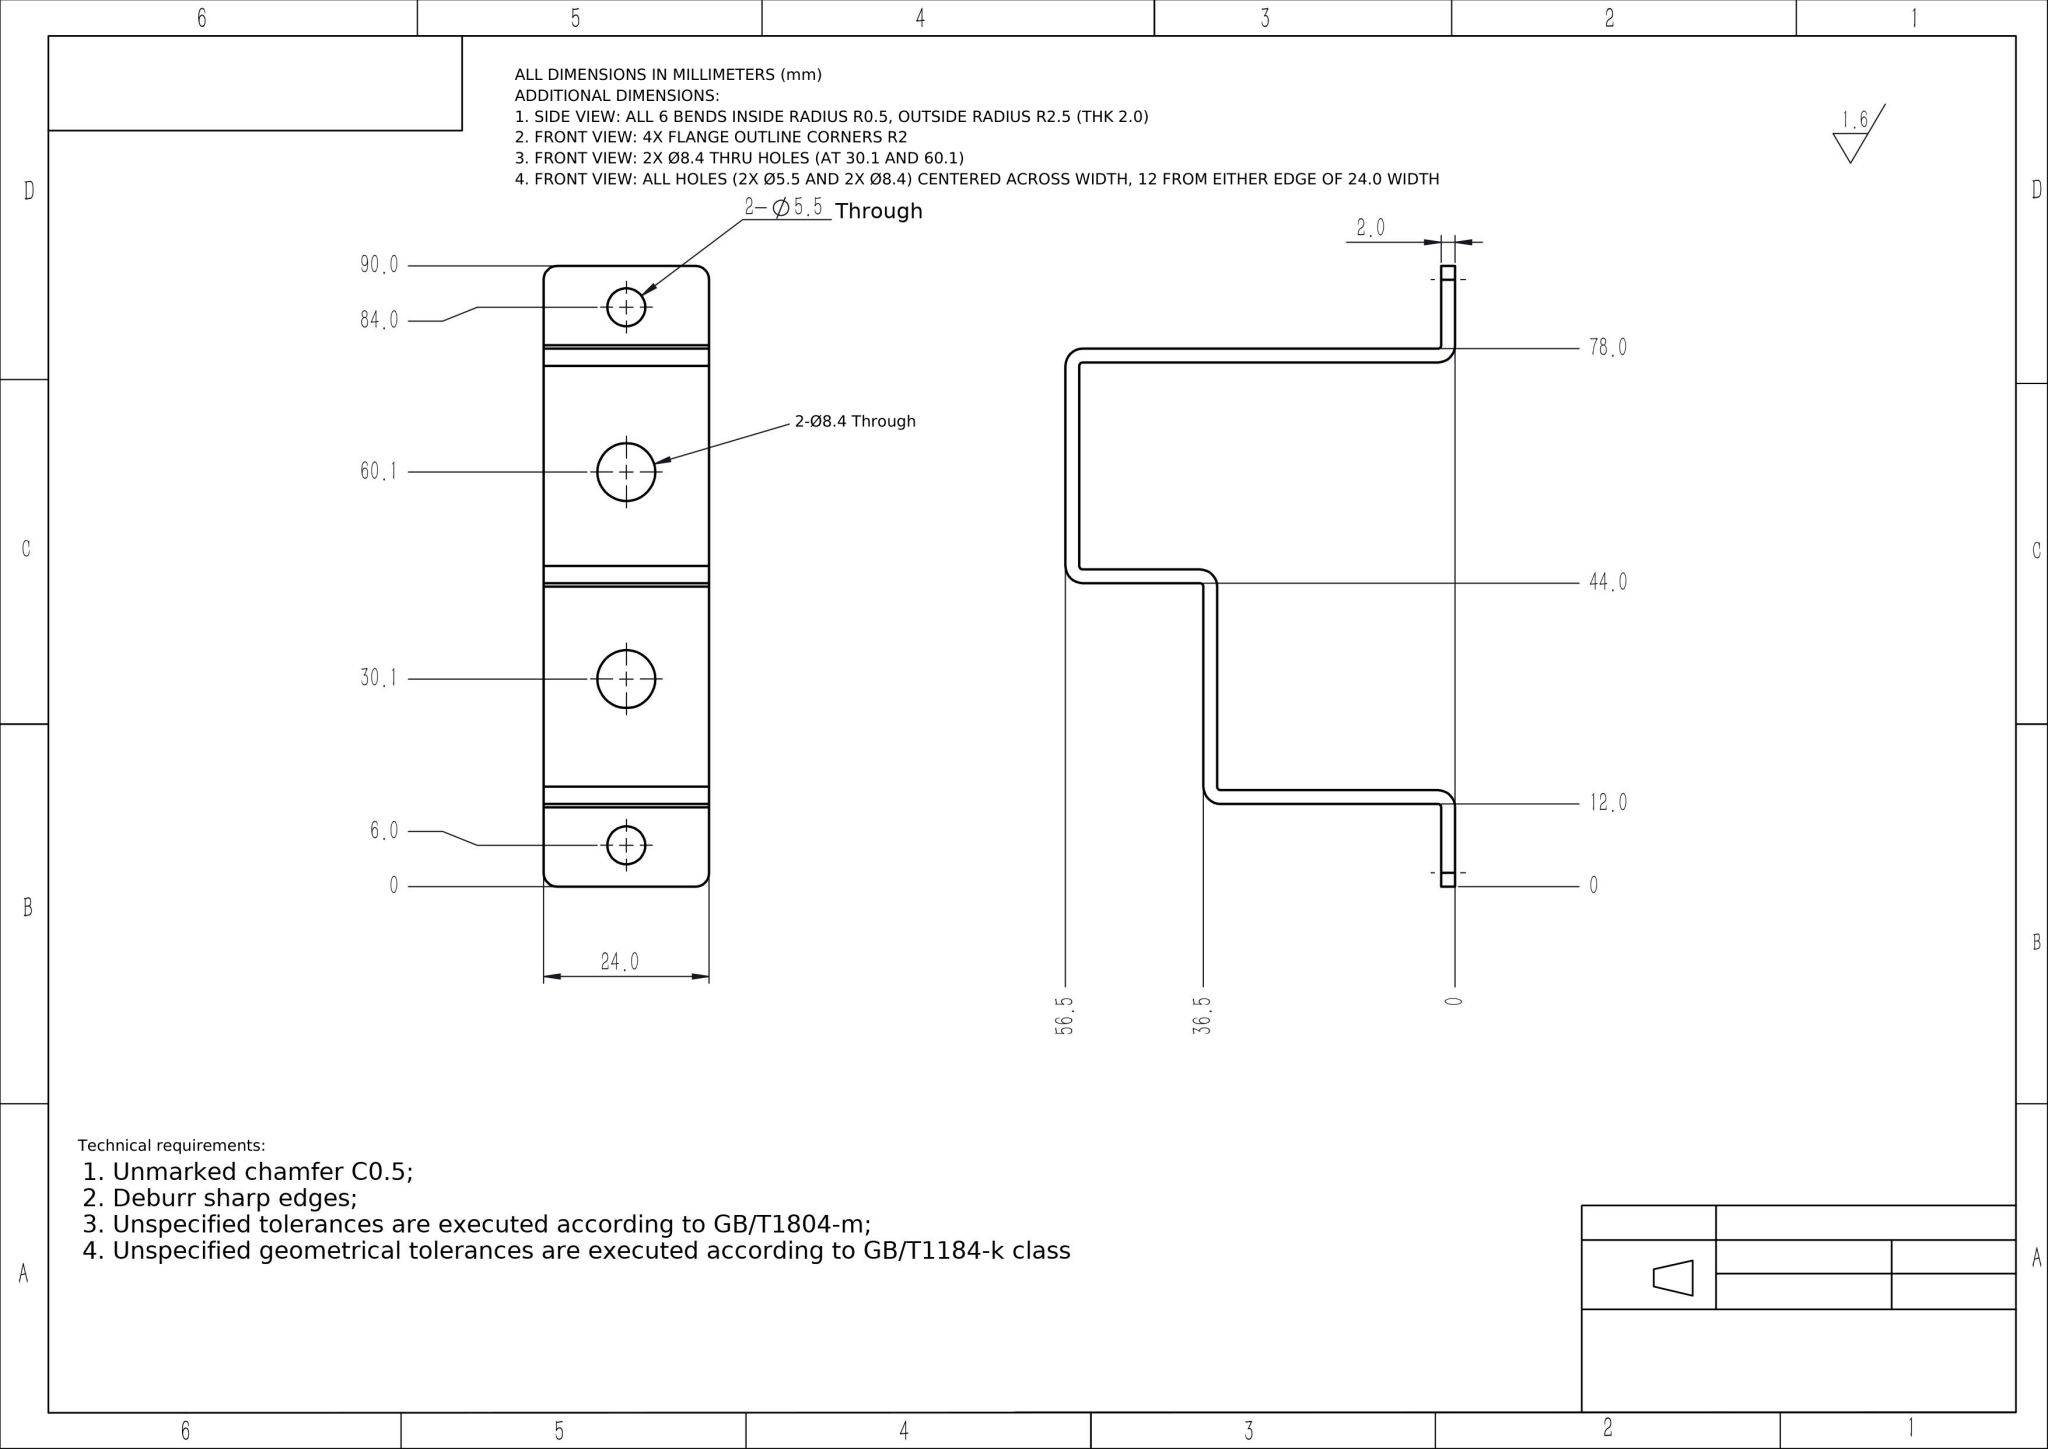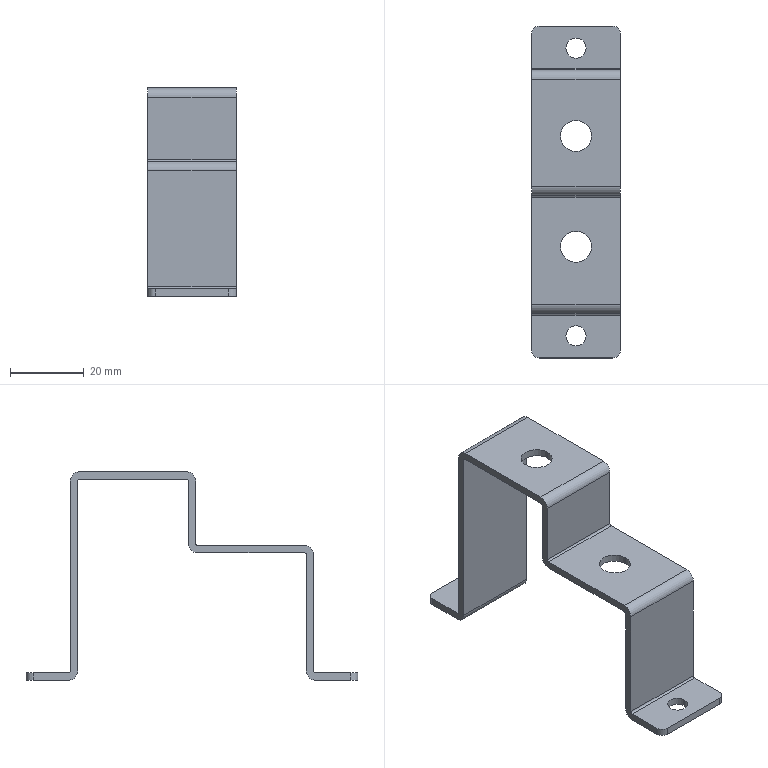Part | NX | mm | 1 solid | 42 faces | box 24 x 90 x 56.5 mm | volume 9043 mm3 | cylinder 24 | plane 18 | commonest cylinder face diameters 1 x6 5 x6 5.5 x4 8.4 x4 4 x4